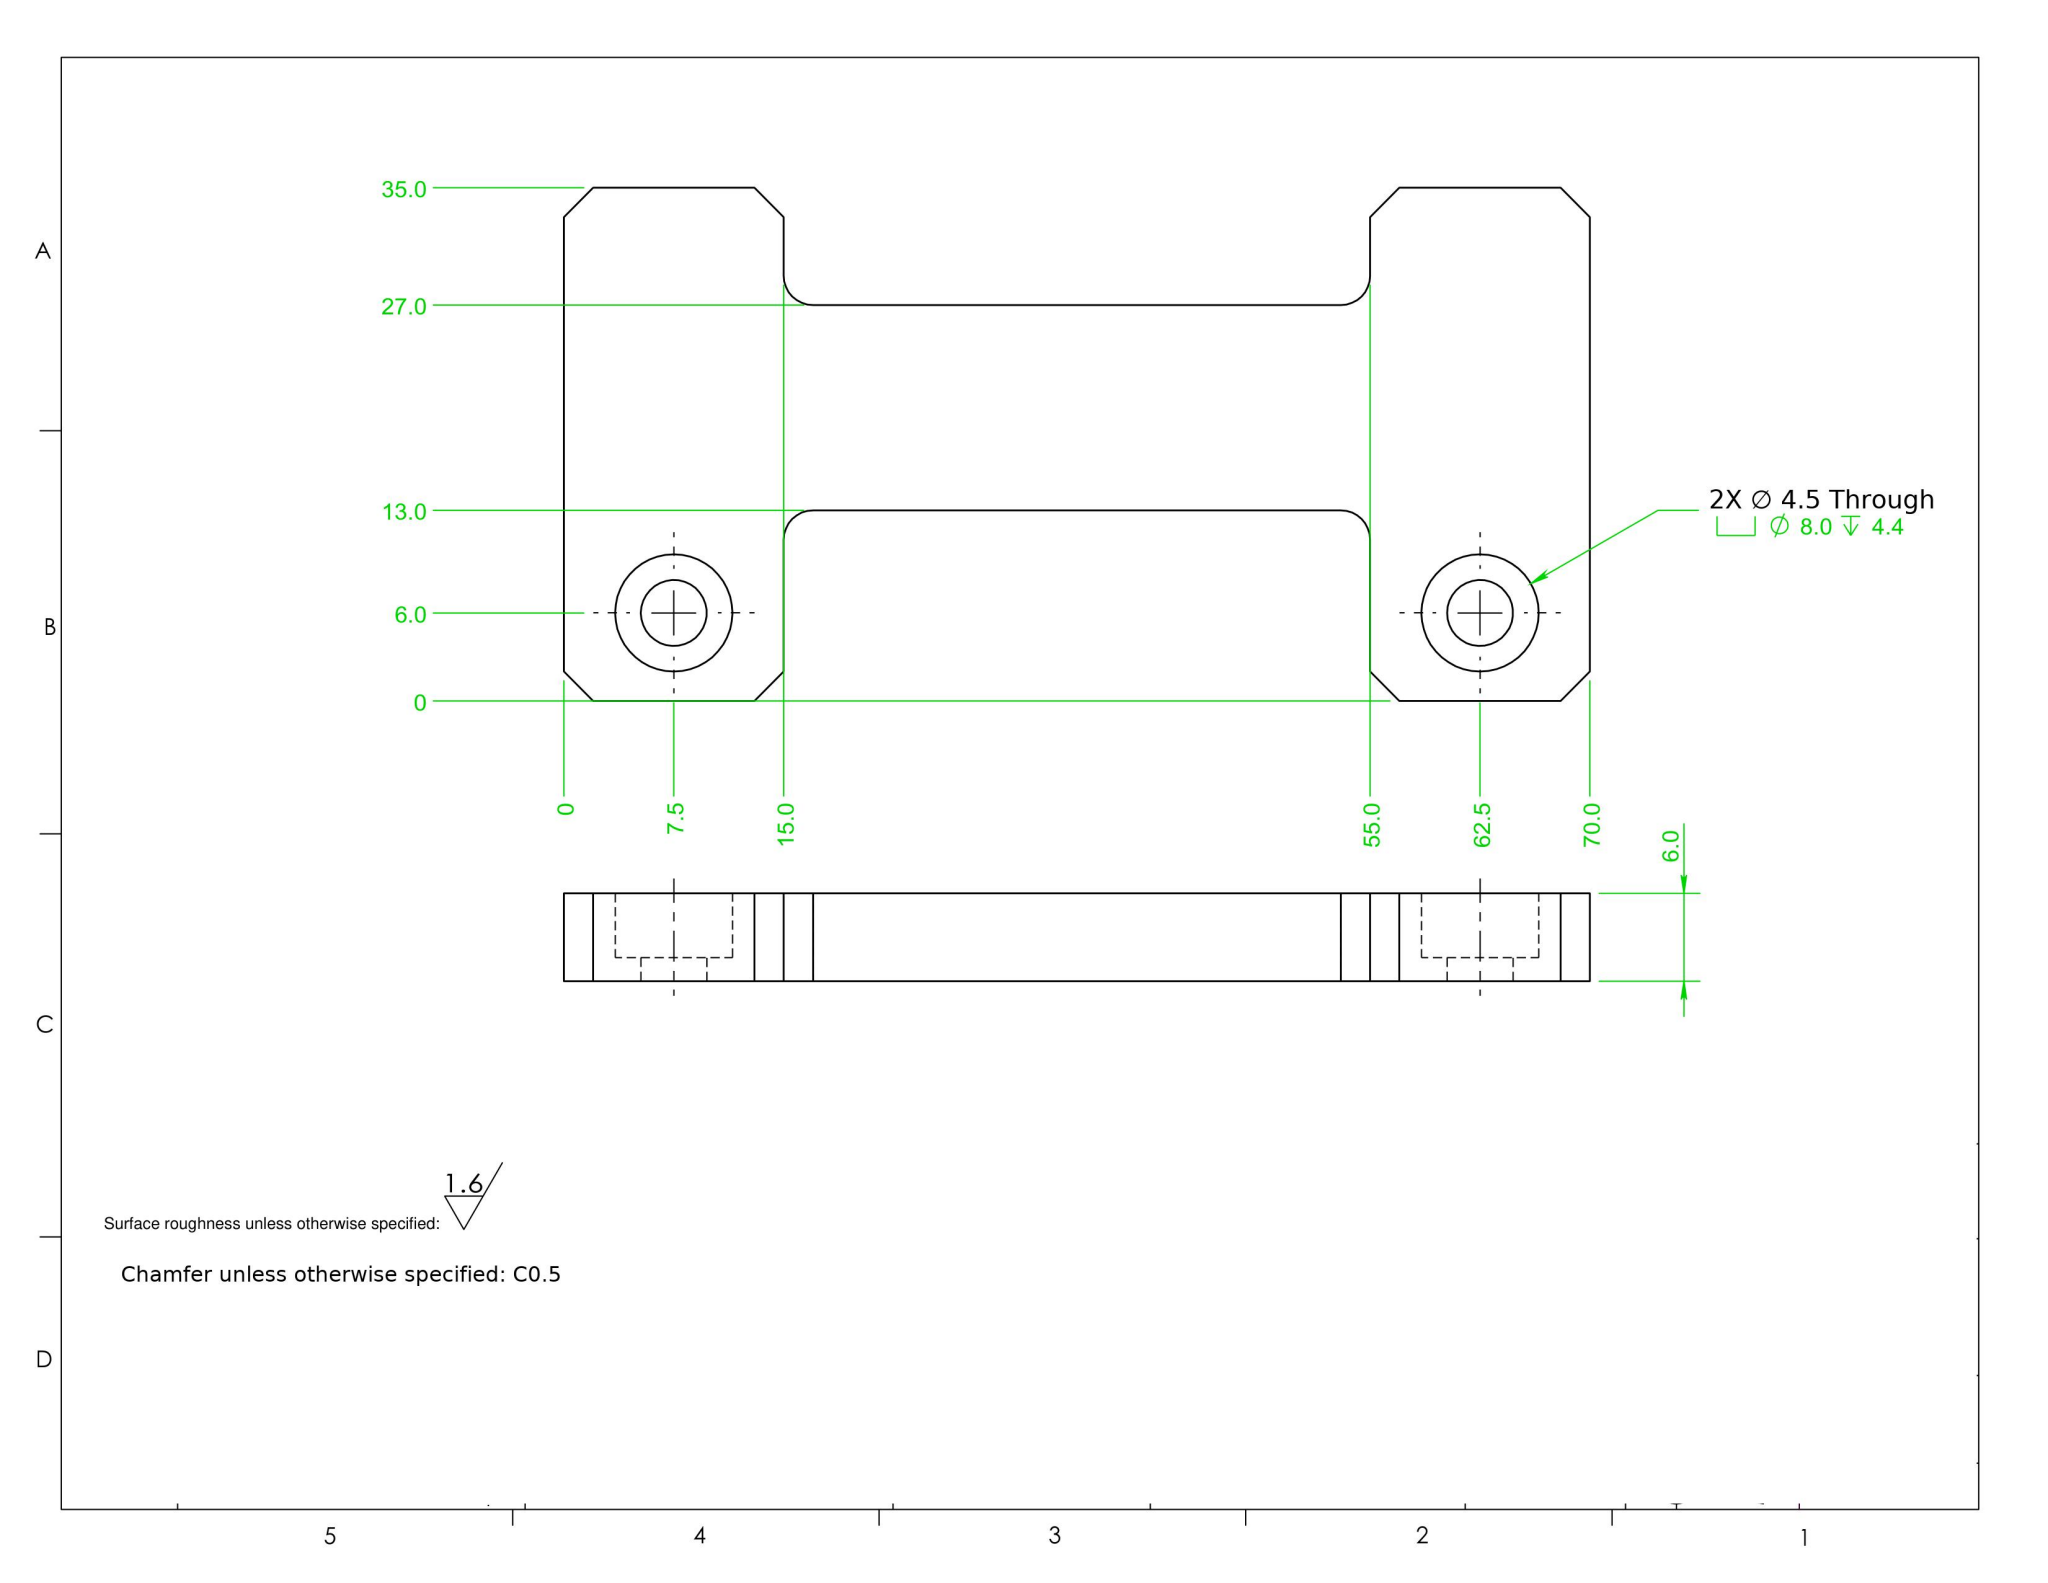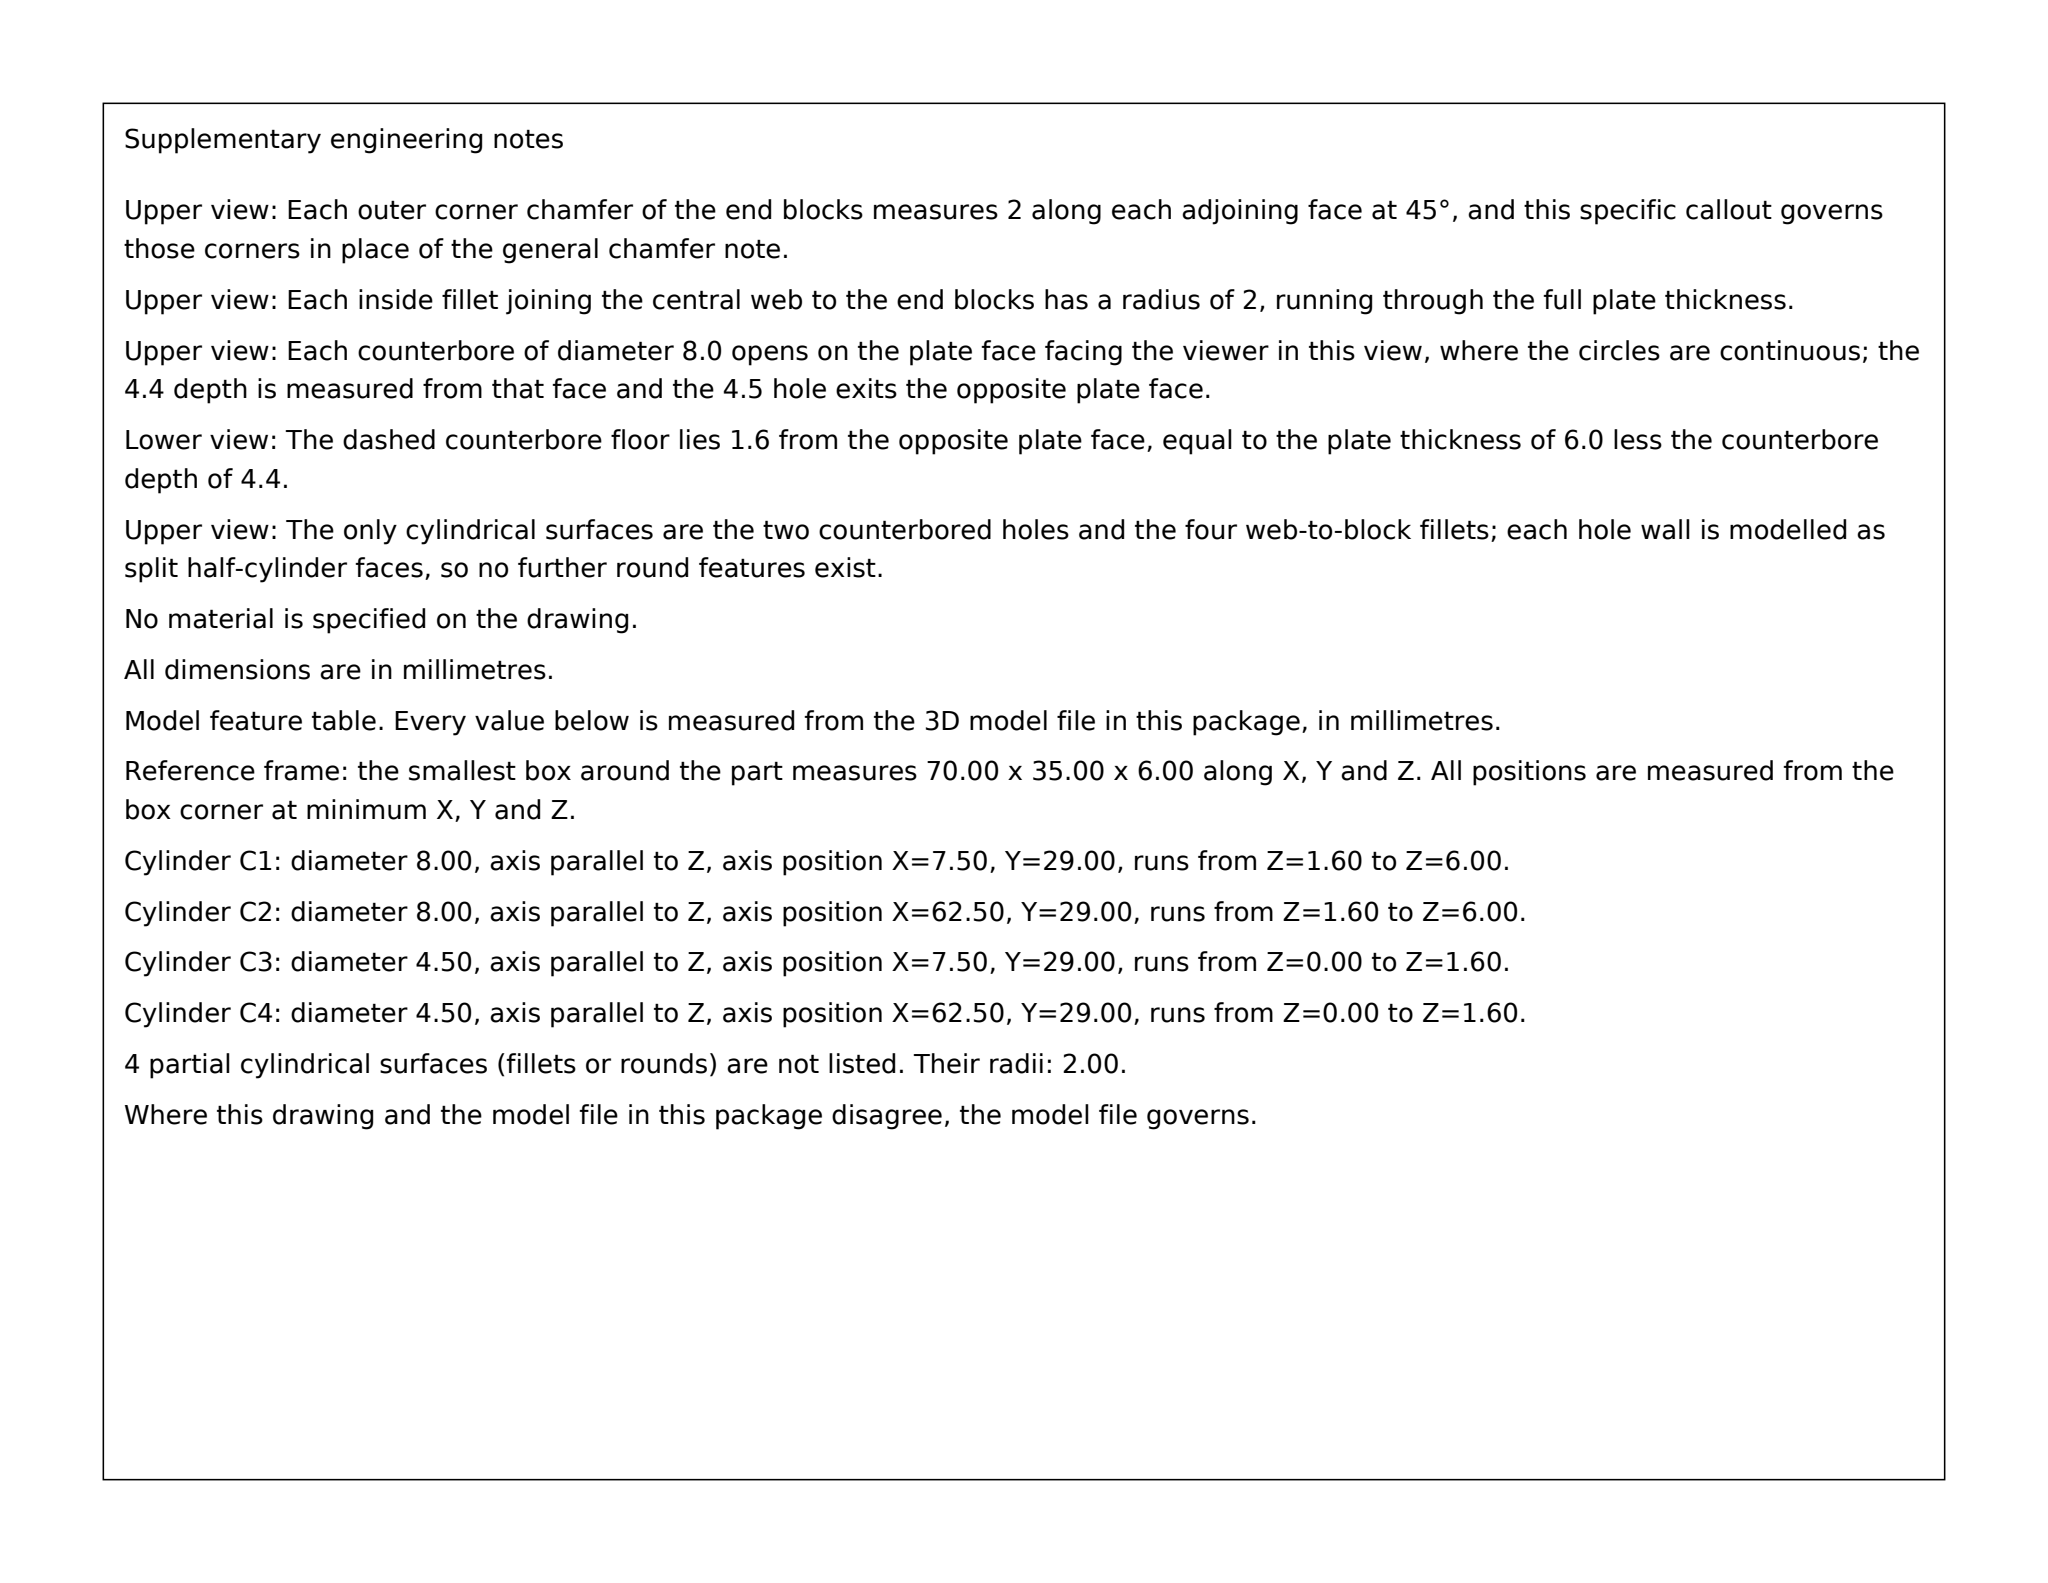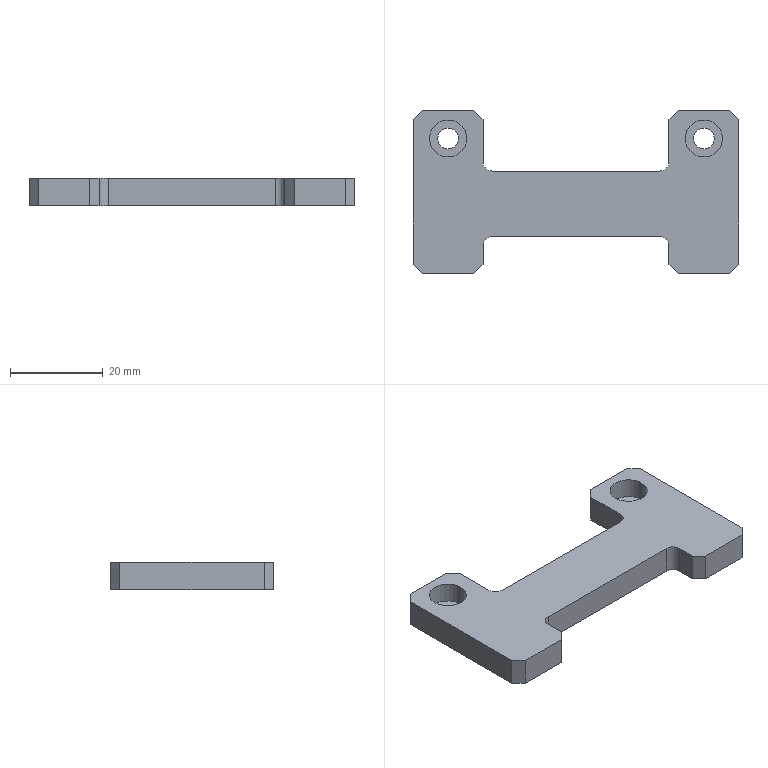Part | SolidWorks | mm | 1 solid | 36 faces | box 70 x 35 x 6 mm | volume 9091 mm3 | plane 24 | cylinder 12 | commonest cylinder face diameters 8 x4 4.5 x4 4 x4
build123d program:
from build123d import *

# Parameters (mm, degrees)
SKETCH1_W                                       = 70
SKETCH1_H                                       = 35
BOSS_EXTRUDE1_DEPTH                             = 6
SKETCH2_W                                       = 40
SKETCH2_H                                       = 13
SKETCH2_H_2                                     = 8
CUT_EXTRUDE1_DEPTH                              = 79.492
M4_HEX_SOCKET_HEAD_CAP_SCREW_CBORE1_D           = 4.5
M4_HEX_SOCKET_HEAD_CAP_SCREW_CBORE1_CBORE_D     = 8
M4_HEX_SOCKET_HEAD_CAP_SCREW_CBORE1_CBORE_DEPTH = 4.4
FILLET1_R                                       = 2
CHAMFER1_SIZE                                   = 2


with BuildPart() as part:
    # Sketch1 → Boss-Extrude1 (new body)
    with BuildSketch(Plane.XY):
        with Locations((35, 17.5)):
            Rectangle(SKETCH1_W, SKETCH1_H)
    extrude(amount=BOSS_EXTRUDE1_DEPTH)

    # Sketch2 → Cut-Extrude1 (cut, through all)
    with BuildSketch(Plane.XY.offset(6)):
        with Locations((35, 28.5)):
            Rectangle(SKETCH2_W, SKETCH2_H)
        with Locations((35, 4)):
            Rectangle(SKETCH2_W, SKETCH2_H_2)
    extrude(amount=-CUT_EXTRUDE1_DEPTH, mode=Mode.SUBTRACT)

    # M4 Hex Socket Head Cap Screw CBORE1 (through all)
    with Locations(Plane.XY.offset(6)):
        with Locations((7.5, 29), (62.5, 29)):
            CounterBoreHole(M4_HEX_SOCKET_HEAD_CAP_SCREW_CBORE1_D / 2, M4_HEX_SOCKET_HEAD_CAP_SCREW_CBORE1_CBORE_D / 2, M4_HEX_SOCKET_HEAD_CAP_SCREW_CBORE1_CBORE_DEPTH)

    # Fillet1
    fillet1_edges = [part.edges().sort_by_distance(p)[0] for p in [
        (15, 22, 3),
        (55, 22, 3),
        (15, 8, 3),
        (55, 8, 3),
    ]]
    fillet(fillet1_edges, radius=FILLET1_R)

    # Chamfer1
    chamfer1_edges = [part.edges().sort_by_distance(p)[0] for p in [
        (15, 35, 3),
        (55, 35, 3),
        (15, 0, 3),
        (55, 0, 3),
        (0, 35, 3),
        (70, 35, 3),
        (70, 0, 3),
        (0, 0, 3),
    ]]
    chamfer(chamfer1_edges, length=CHAMFER1_SIZE)


solid = part.part